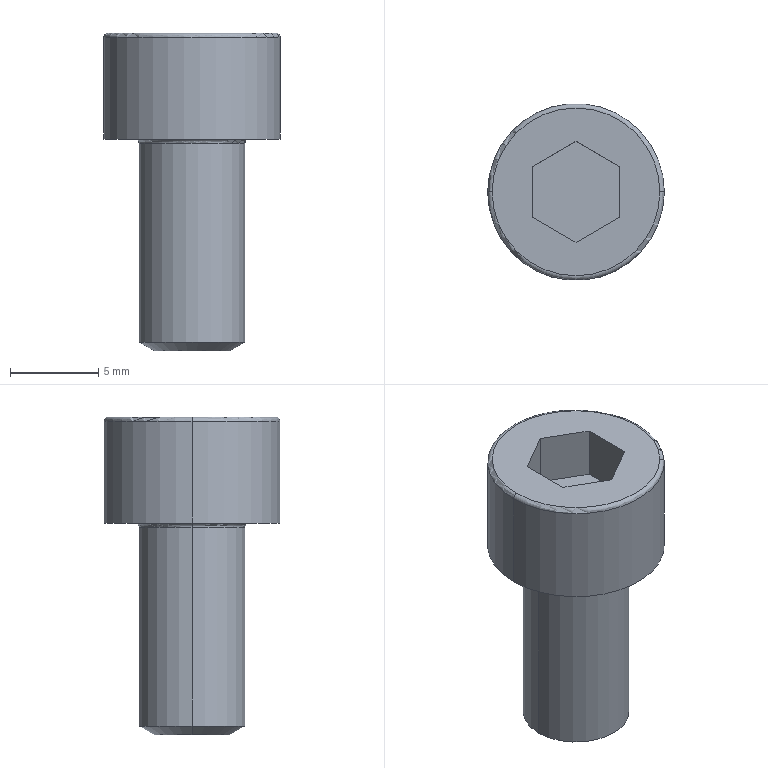Component | NX | SHCS_M6X12 | 1 solid | 20 faces | volume 743 mm3 | plane 10 | torus 4 | cylinder 4 | cone 2 | commonest cylinder face diameters 10 x2 6 x2